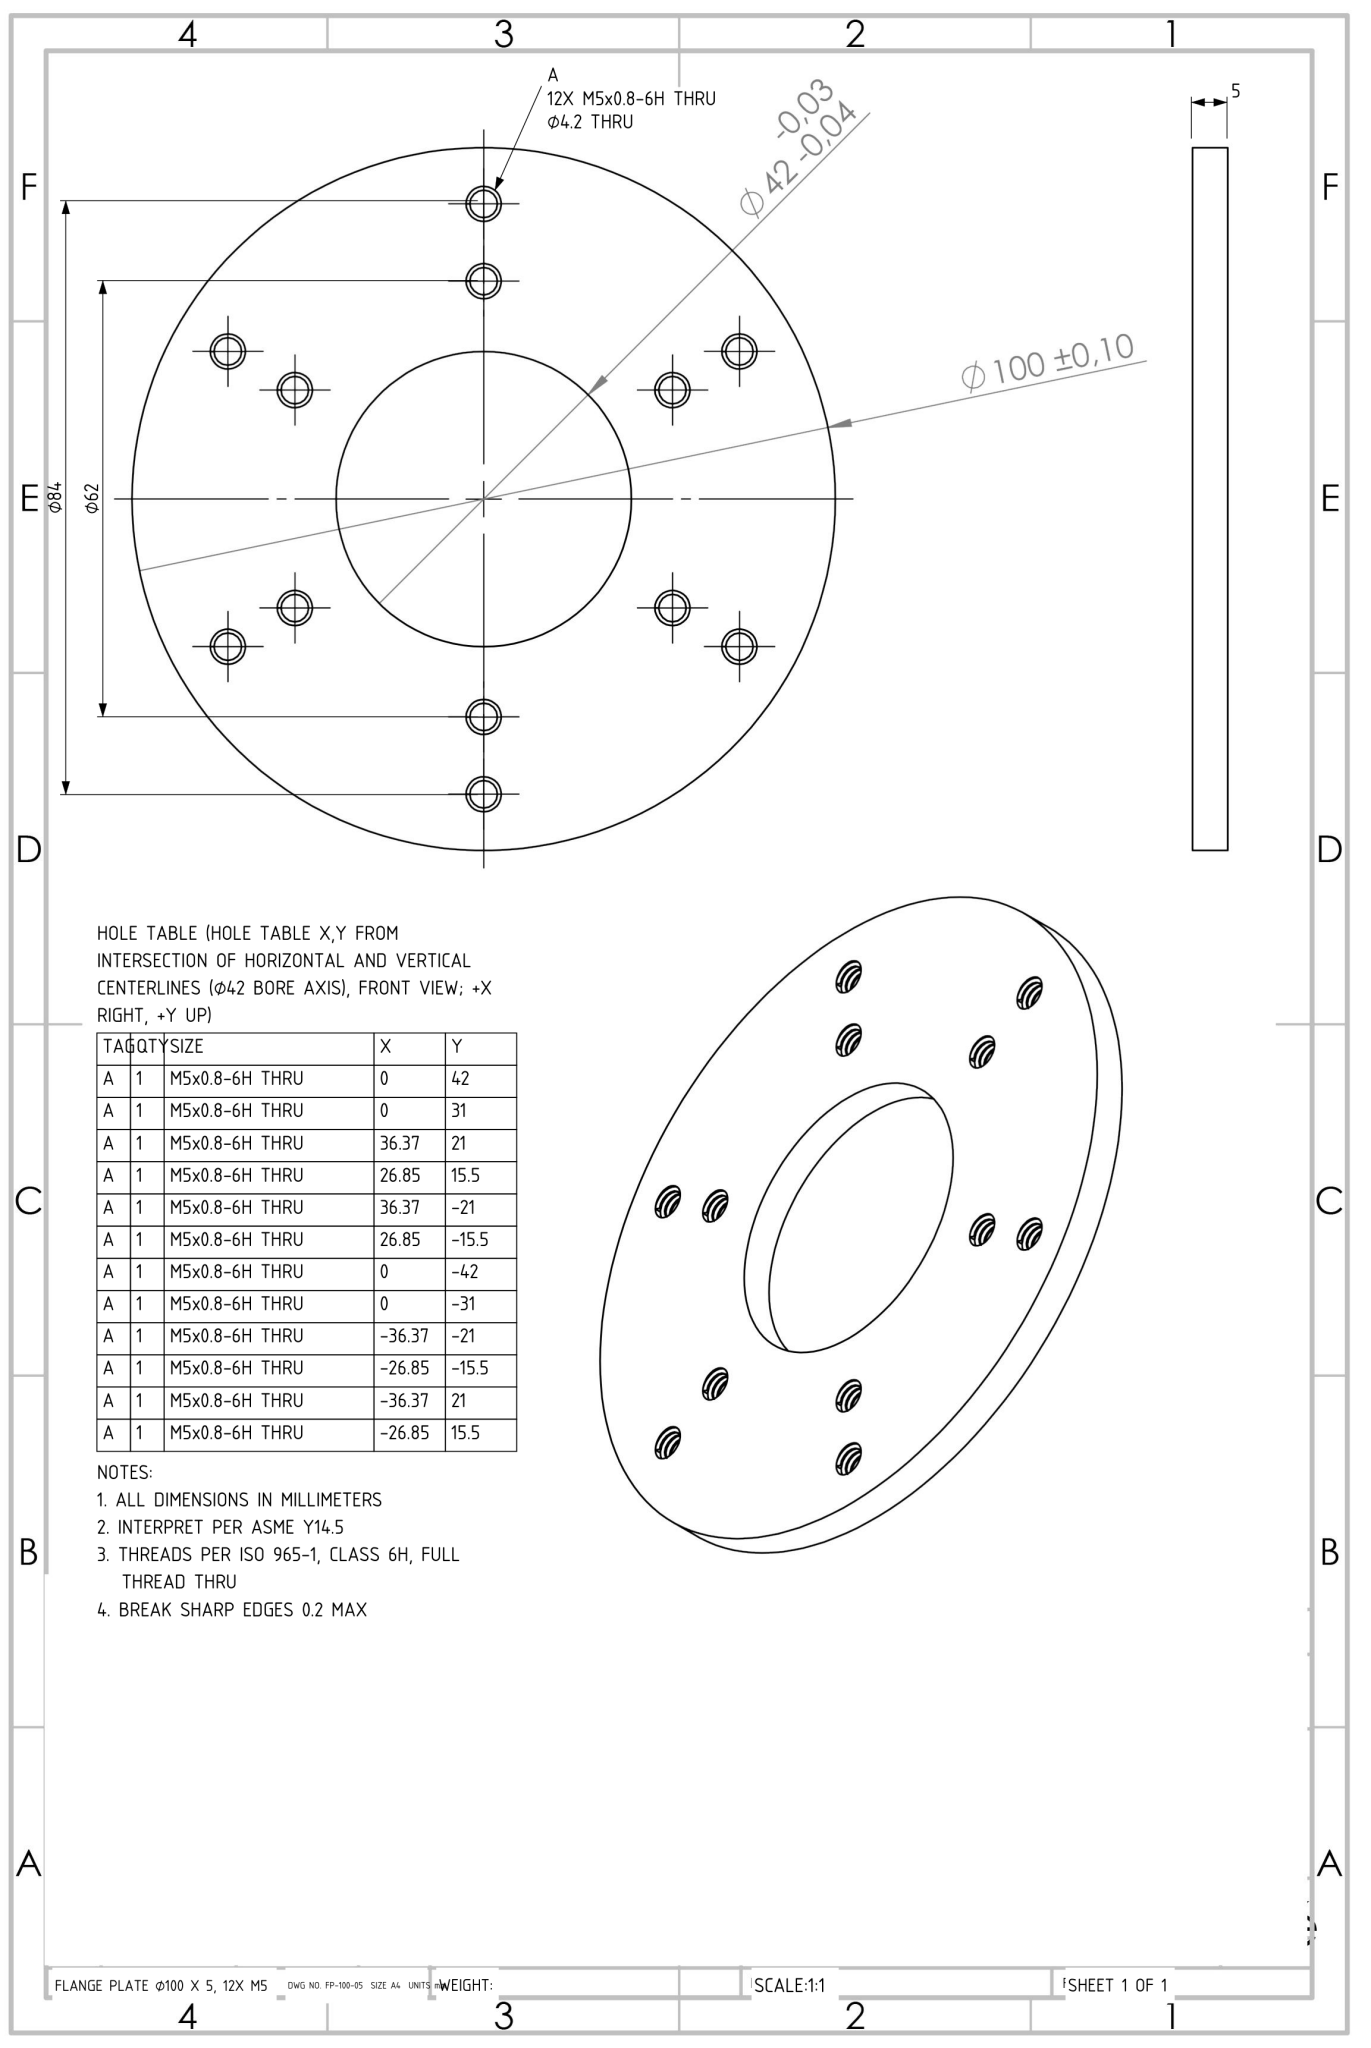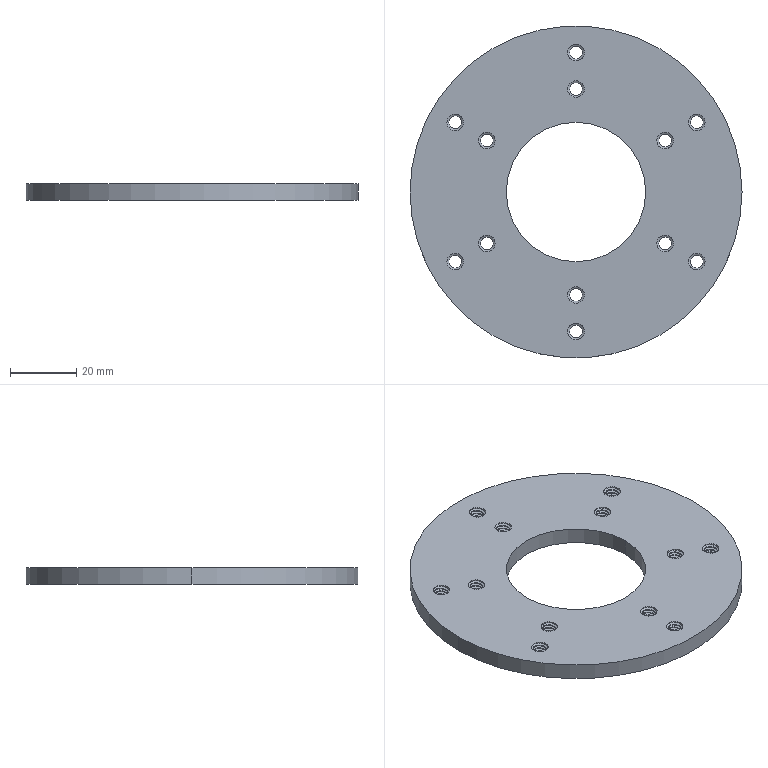Part | NX | mm | 1 solid | 186 faces | box 100 x 100 x 5 mm | volume 31374 mm3 | cylinder 124 | spline 36 | plane 26 | commonest cylinder face diameters 5 x120 42 x2 100 x2